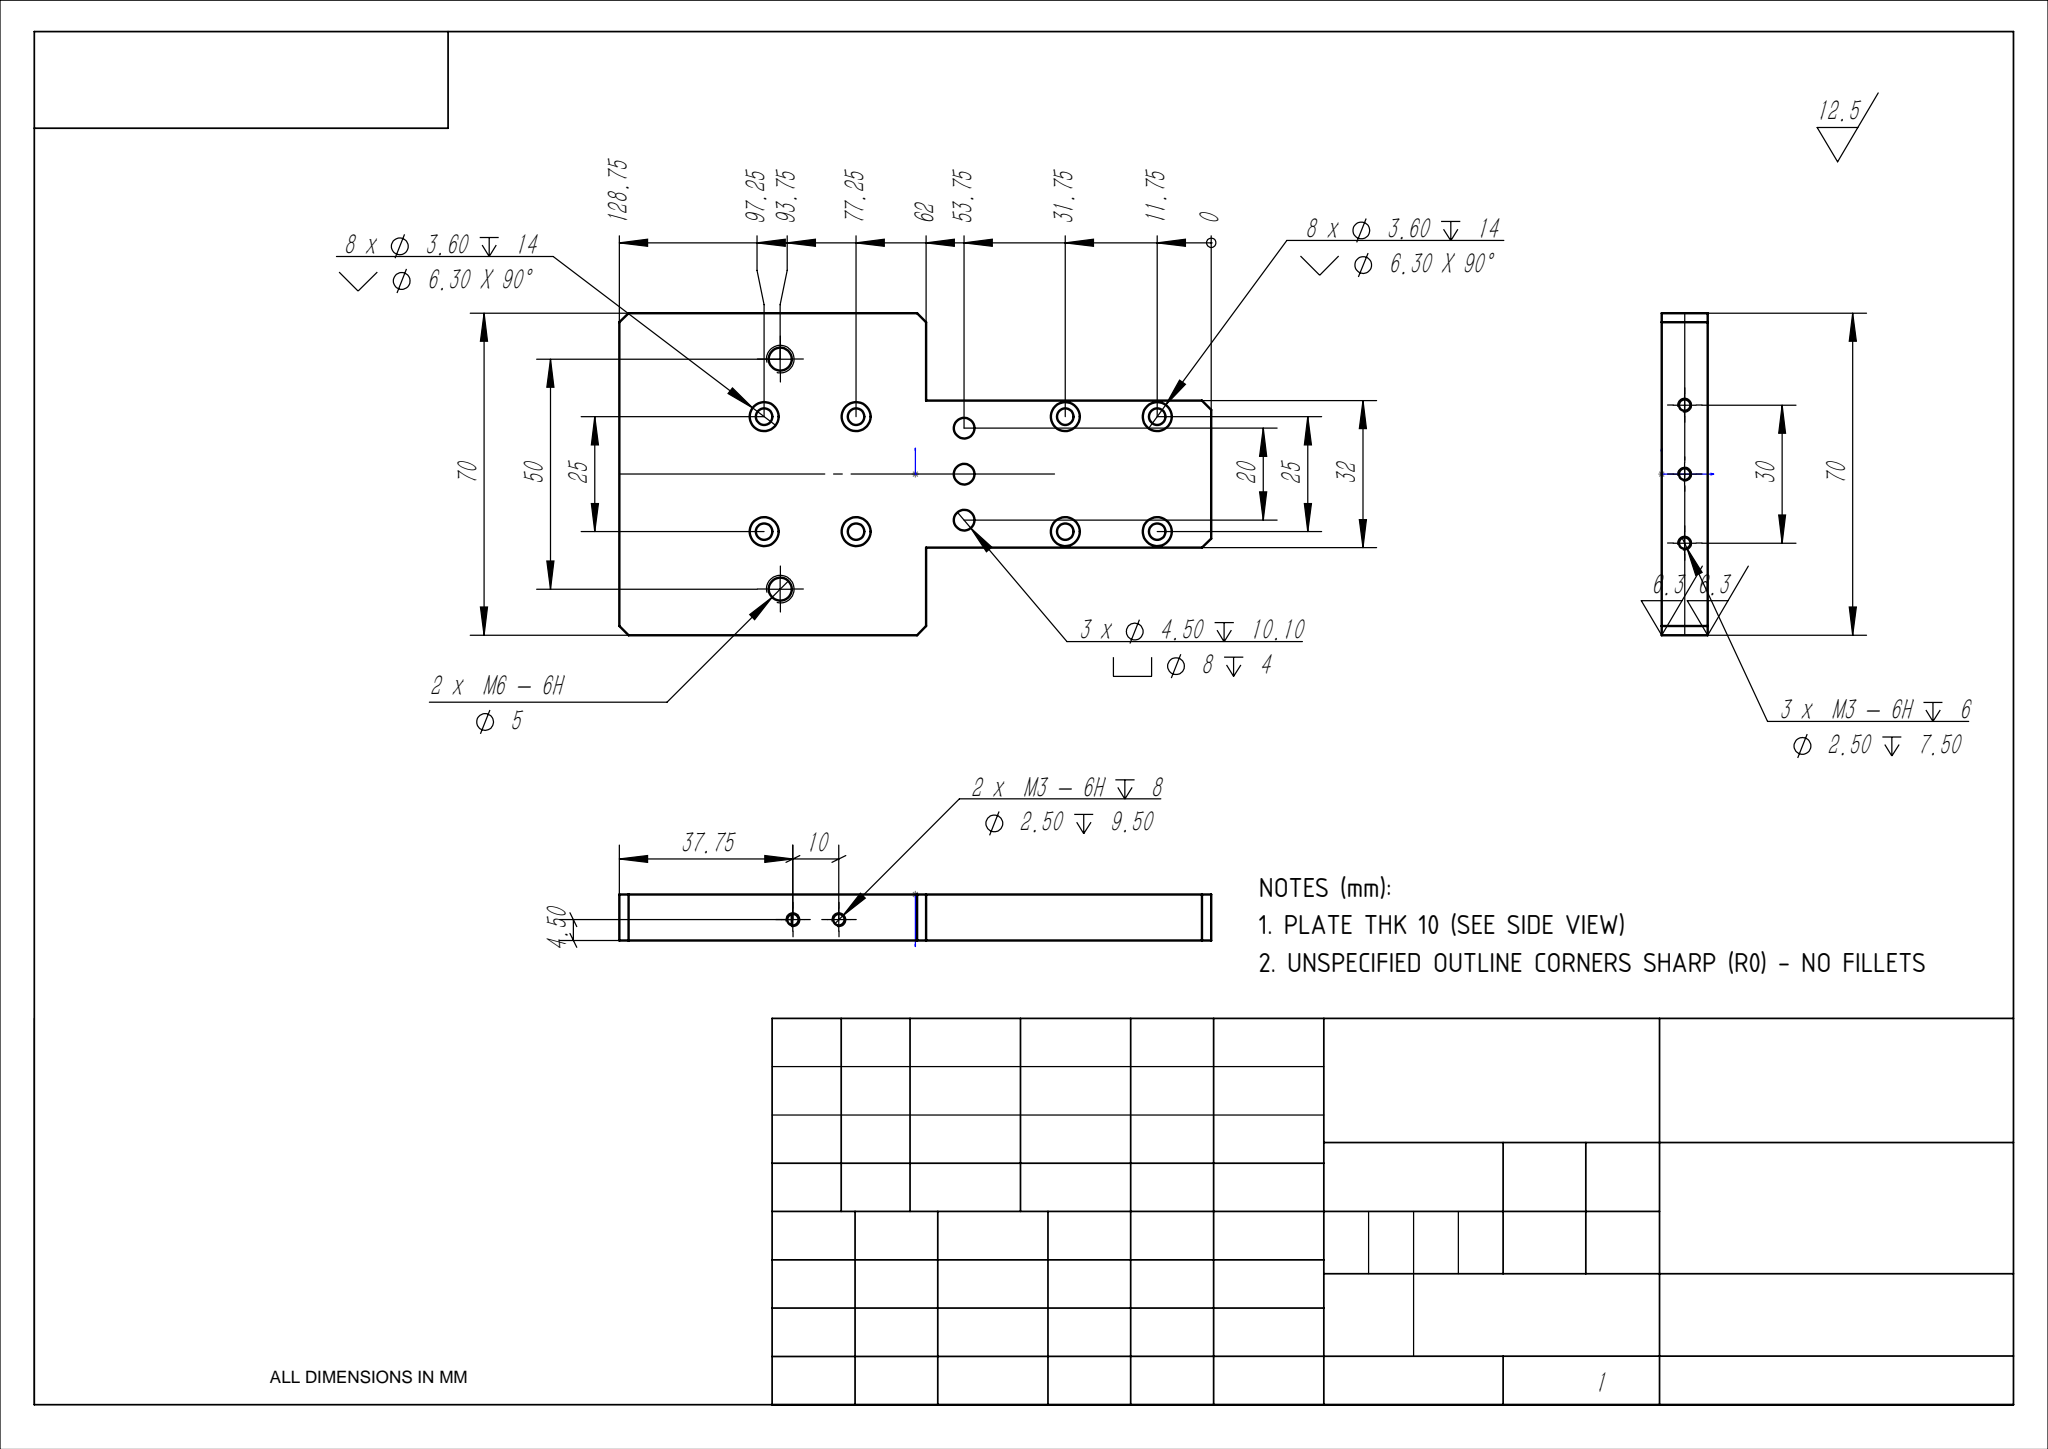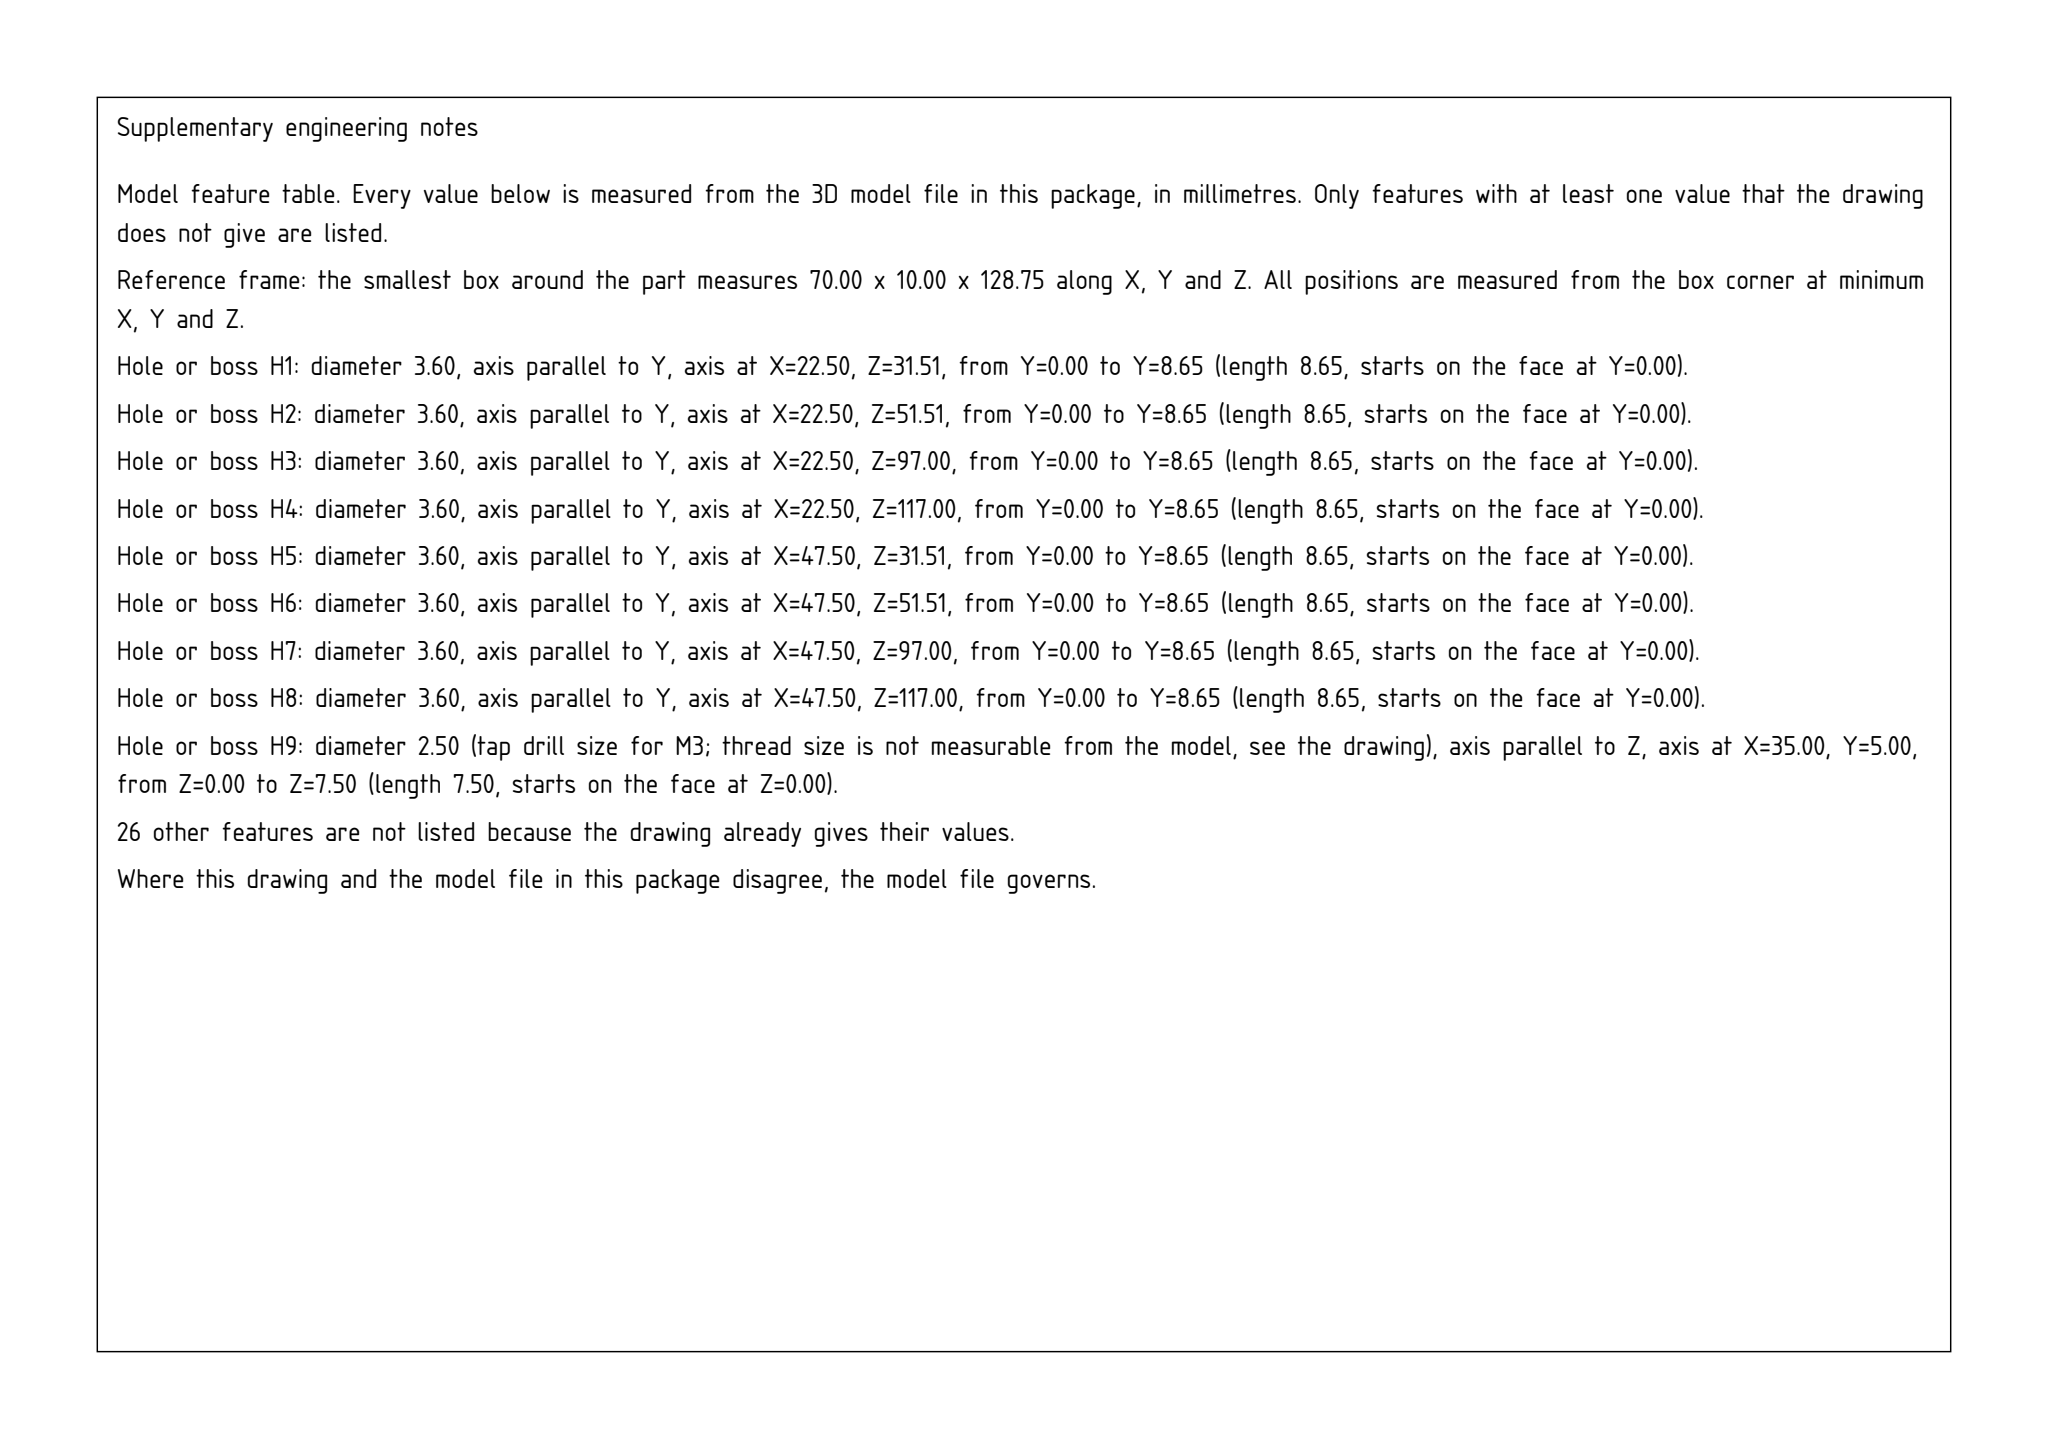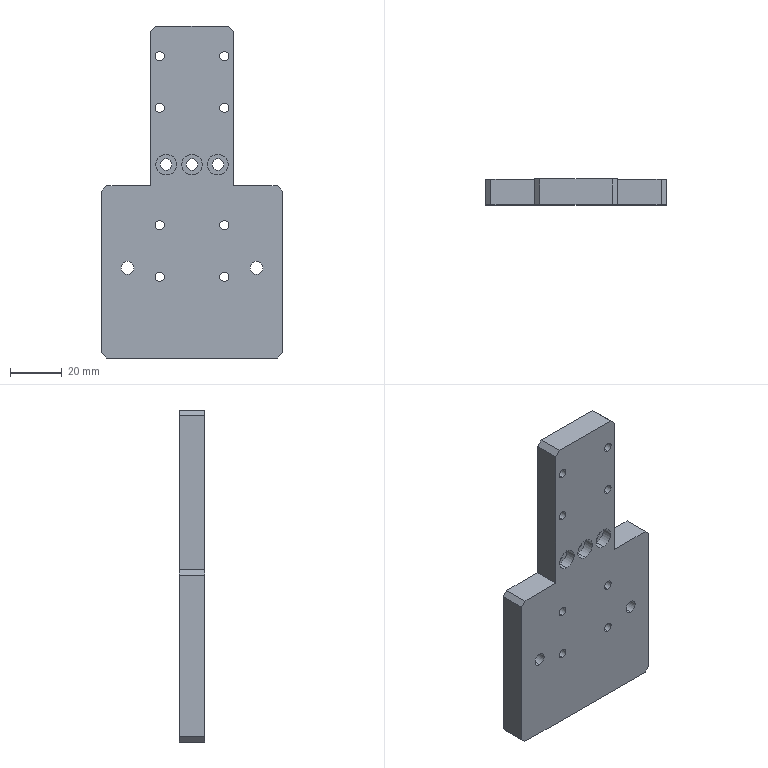Part | SolidWorks | mm | 1 solid | 87 faces | box 70 x 10 x 128.75 mm | volume 64037 mm3 | cylinder 42 | cone 26 | plane 19 | commonest cylinder face diameters 3.6 x16 2.5 x10 8 x6 4.5 x6 5 x4
Drawing notes:
PLATE THK 10 (SEE SIDE VIEW) | from the solid: bbox_xyz y = 10.0; faces y=0.0 and y=10.0 bound plate
UNSPECIFIED OUTLINE CORNERS SHARP (R0) - NO FILLETS | from the solid: fillet_radii: [] ; outline formed only by planar faces (x=0,19,51,70; z=0,66.75,128.75)
build123d program:
from build123d import *

# Parameters (mm, degrees)
SKETCH1_W                                            = 70
SKETCH1_H                                            = 128.75
BOSS_EXTRUDE1_DEPTH                                  = 10
M6_TAPPED_HOLE1_D                                    = 5
CHAMFER1_SIZE                                        = 5
M3_FLAT_HEAD_MACHINE_SCREW_TAPERED_COUNT_D           = 3.6
M3_FLAT_HEAD_MACHINE_SCREW_TAPERED_COUNT_DEPTH       = 14
M3_FLAT_HEAD_MACHINE_SCREW_TAPERED_COUNT_CSINK_D     = 6.3
M3_FLAT_HEAD_MACHINE_SCREW_TAPERED_COUNT_CSINK_ANGLE = 90
SKETCH12_W                                           = 19
SKETCH12_H                                           = 62
CUT_EXTRUDE1_DEPTH                                   = 10
M3_TAPPED_HOLE2_D                                    = 2.5
M3_TAPPED_HOLE2_DEPTH                                = 9.5
M3_TAPPED_HOLE2_TIP                                  = 0.7511
M3_TAPPED_HOLE3_D                                    = 2.5
M3_TAPPED_HOLE3_DEPTH                                = 7.5
M3_TAPPED_HOLE3_TIP                                  = 0.7511
M4_SOCKET_HEAD_CAP_SCREW_CYLINDRICAL_COU_D           = 4.5
M4_SOCKET_HEAD_CAP_SCREW_CYLINDRICAL_COU_DEPTH       = 10.1
M4_SOCKET_HEAD_CAP_SCREW_CYLINDRICAL_COU_CBORE_D     = 8
M4_SOCKET_HEAD_CAP_SCREW_CYLINDRICAL_COU_CBORE_DEPTH = 4
M4_SOCKET_HEAD_CAP_SCREW_CYLINDRICAL_COU_TIP         = 1.352
CHAMFER2_SIZE                                        = 2


with BuildPart() as part:
    # Sketch1 → Boss-Extrude1 (new body)
    with BuildSketch(Plane(origin=(0, 0, 0), x_dir=(1, 0, 0), z_dir=(0, 1, 0))):
        Rectangle(SKETCH1_W, SKETCH1_H)
    extrude(amount=BOSS_EXTRUDE1_DEPTH)

    # M6 Tapped Hole1 (through all)
    with Locations(Plane(origin=(0, 10, 0), x_dir=(1, 0, 0), z_dir=(0, 1, 0))):
        with Locations((-25, 29.375), (25, 29.375)):
            Hole(M6_TAPPED_HOLE1_D / 2)

    # Chamfer1
    chamfer1_edges = [part.edges().sort_by_distance(p)[0] for p in [
        (35, 5, 64.375),
        (-35, 5, 64.375),
    ]]
    chamfer(chamfer1_edges, length=CHAMFER1_SIZE)

    # M3 Flat Head Machine Screw Tapered Count
    with Locations(Plane(origin=(0, 10, 0), x_dir=(1, 0, 0), z_dir=(0, 1, 0))):
        with Locations((-12.5, 32.875), (-12.5, 12.875), (12.5, 32.875), (12.5, 12.875), (-12.5, -32.625), (-12.5, -52.625), (12.5, -32.625), (12.5, -52.625)):
            CounterSinkHole(M3_FLAT_HEAD_MACHINE_SCREW_TAPERED_COUNT_D / 2, M3_FLAT_HEAD_MACHINE_SCREW_TAPERED_COUNT_CSINK_D / 2, depth=M3_FLAT_HEAD_MACHINE_SCREW_TAPERED_COUNT_DEPTH, counter_sink_angle=M3_FLAT_HEAD_MACHINE_SCREW_TAPERED_COUNT_CSINK_ANGLE)

    # Sketch12 → Cut-Extrude1 (cut)
    with BuildSketch(Plane(origin=(0, 10, 0), x_dir=(1, 0, 0), z_dir=(0, 1, 0))):
        with Locations((-25.5, -33.375)):
            Rectangle(SKETCH12_W, SKETCH12_H)
        with Locations((25.5, -33.375)):
            Rectangle(SKETCH12_W, SKETCH12_H)
    extrude(amount=-CUT_EXTRUDE1_DEPTH, mode=Mode.SUBTRACT)

    # M3 Tapped Hole2
    with Locations(Plane(origin=(35, 0, 0), x_dir=(0, 0, -1), z_dir=(1, 0, 0))):
        with Locations((16.625, 5.5), (26.625, 5.5)):
            Hole(M3_TAPPED_HOLE2_D / 2, depth=M3_TAPPED_HOLE2_DEPTH)
            with Locations((0, 0, -(M3_TAPPED_HOLE2_DEPTH + M3_TAPPED_HOLE2_TIP / 2))):  # 118° drill point
                Cone(0, M3_TAPPED_HOLE2_D / 2, M3_TAPPED_HOLE2_TIP, mode=Mode.SUBTRACT)

    # M3 Tapped Hole3
    with Locations(Plane(origin=(0, 0, -64.375), x_dir=(-1, 0, 0), z_dir=(0, 0, -1))):
        with Locations((-15, 5), (0, 5), (15, 5)):
            Hole(M3_TAPPED_HOLE3_D / 2, depth=M3_TAPPED_HOLE3_DEPTH)
            with Locations((0, 0, -(M3_TAPPED_HOLE3_DEPTH + M3_TAPPED_HOLE3_TIP / 2))):  # 118° drill point
                Cone(0, M3_TAPPED_HOLE3_D / 2, M3_TAPPED_HOLE3_TIP, mode=Mode.SUBTRACT)

    # M4 Socket Head Cap Screw Cylindrical Cou
    with Locations(Plane(origin=(0, 0, 0), x_dir=(-1, 0, 0), z_dir=(0, -1, 0))):
        with Locations((10, -10.625), (0, -10.625), (-10, -10.625)):
            CounterBoreHole(M4_SOCKET_HEAD_CAP_SCREW_CYLINDRICAL_COU_D / 2, M4_SOCKET_HEAD_CAP_SCREW_CYLINDRICAL_COU_CBORE_D / 2, M4_SOCKET_HEAD_CAP_SCREW_CYLINDRICAL_COU_CBORE_DEPTH, depth=M4_SOCKET_HEAD_CAP_SCREW_CYLINDRICAL_COU_DEPTH)
            with Locations((0, 0, -(M4_SOCKET_HEAD_CAP_SCREW_CYLINDRICAL_COU_DEPTH + M4_SOCKET_HEAD_CAP_SCREW_CYLINDRICAL_COU_TIP / 2))):  # 118° drill point
                Cone(0, M4_SOCKET_HEAD_CAP_SCREW_CYLINDRICAL_COU_D / 2, M4_SOCKET_HEAD_CAP_SCREW_CYLINDRICAL_COU_TIP, mode=Mode.SUBTRACT)

    # Chamfer2
    chamfer2_edges = [part.edges().sort_by_distance(p)[0] for p in [
        (-35, 5, 2.375),
        (-16, 5, 64.375),
        (35, 5, 2.375),
        (16, 5, 64.375),
        (-35, 5, -64.375),
        (35, 5, -64.375),
    ]]
    chamfer(chamfer2_edges, length=CHAMFER2_SIZE)


solid = part.part